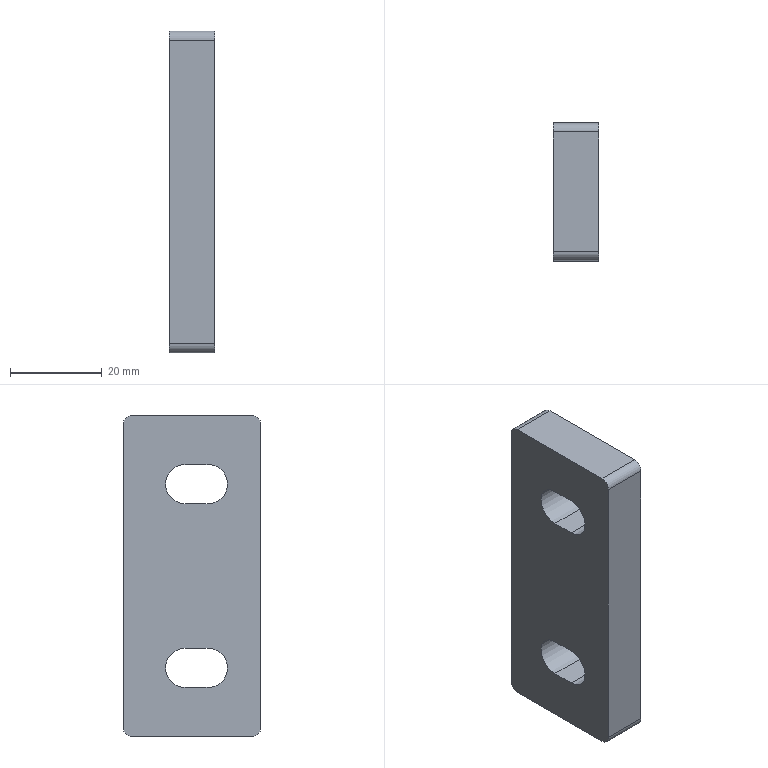Component | SolidWorks | BladeHolderPlate.1-2 | 1 solid | 26 faces | box 10 x 30 x 70 mm | volume 18626 mm3 | cylinder 12 | plane 10 | cone 4 | commonest cylinder face diameters 4.2 x4 4 x4 8.5 x4
build123d program:
from build123d import *

# Parameters (mm, degrees)
BOSS_EXTRUDE1_DEPTH   = 10
M5_TAPPED_HOLE1_D     = 4.2
M5_TAPPED_HOLE1_DEPTH = 12.4
M5_TAPPED_HOLE1_TIP   = 1.262
CUT_EXTRUDE1_DEPTH    = 15


with BuildPart() as part:
    # Sketch1 → Boss-Extrude1 (new body)
    with BuildSketch(Plane.XY):
        with BuildLine():
            Line((-33, 15), (33, 15))
            ThreePointArc((33, 15), (34.414, 14.414), (35, 13))
            Line((35, 13), (35, -13))
            ThreePointArc((35, -13), (34.414, -14.414), (33, -15))
            Line((33, -15), (-33, -15))
            ThreePointArc((-33, -15), (-34.414, -14.414), (-35, -13))
            Line((-35, -13), (-35, 13))
            ThreePointArc((-35, 13), (-34.414, 14.414), (-33, 15))
        make_face()
    extrude(amount=BOSS_EXTRUDE1_DEPTH)

    # M5 Tapped Hole1
    with Locations(Plane(origin=(0, 15, 0), x_dir=(-1, 0, 0), z_dir=(0, 1, 0))):
        with Locations((27.5, 5), (-27.5, 5)):
            Hole(M5_TAPPED_HOLE1_D / 2, depth=M5_TAPPED_HOLE1_DEPTH)
            with Locations((0, 0, -(M5_TAPPED_HOLE1_DEPTH + M5_TAPPED_HOLE1_TIP / 2))):  # 118° drill point
                Cone(0, M5_TAPPED_HOLE1_D / 2, M5_TAPPED_HOLE1_TIP, mode=Mode.SUBTRACT)

    # Sketch5 → Cut-Extrude1 (cut)
    with BuildSketch(Plane.XY.offset(10)):
        with BuildLine():
            Line((-15.75, 1.5), (-15.75, -3.5))
            ThreePointArc((-15.75, -3.5), (-20, -7.75), (-24.25, -3.5))
            Line((-24.25, -3.5), (-24.25, 1.5))
            ThreePointArc((-24.25, 1.5), (-20, 5.75), (-15.75, 1.5))
        make_face()
        with BuildLine():
            Line((24.25, 1.5), (24.25, -3.5))
            ThreePointArc((24.25, -3.5), (20, -7.75), (15.75, -3.5))
            Line((15.75, -3.5), (15.75, 1.5))
            ThreePointArc((15.75, 1.5), (20, 5.75), (24.25, 1.5))
        make_face()
    extrude(amount=-CUT_EXTRUDE1_DEPTH, mode=Mode.SUBTRACT)


solid = part.part

# Placed as in the assembly
solid = solid.moved(Location((-27.75, 191, 0), (0, 90, 0)))
STEP:
#1=CARTESIAN_POINT('',(-0.813,7.622,-1.083));
#2=VERTEX_POINT('',#1);
#3=CARTESIAN_POINT('',(-0.9783,7.622,-1.083));
#4=VERTEX_POINT('',#3);
#5=CARTESIAN_POINT('',(-0.8957,7.622,-1.083));
#6=DIRECTION('',(-0.,1.,-0.));
#7=DIRECTION('',(-1.,0.,0.));
#8=AXIS2_PLACEMENT_3D('',#5,#6,#7);
#9=CIRCLE('',#8,0.08268);
#10=EDGE_CURVE('',#2,#4,#9,.T.);
#11=ORIENTED_EDGE('',*,*,#10,.F.);
#12=CARTESIAN_POINT('',(-0.813,8.11,-1.083));
#13=VERTEX_POINT('',#12);
#14=CARTESIAN_POINT('',(-0.813,8.11,-1.083));
#15=DIRECTION('',(-0.,1.,-0.));
#16=VECTOR('',#15,39.37);
#17=LINE('',#14,#16);
#18=EDGE_CURVE('',#2,#13,#17,.T.);
#19=ORIENTED_EDGE('',*,*,#18,.T.);
#20=CARTESIAN_POINT('',(-0.9783,8.11,-1.083));
#21=VERTEX_POINT('',#20);
#22=CARTESIAN_POINT('',(-0.8957,8.11,-1.083));
#23=DIRECTION('',(-0.,1.,-0.));
#24=DIRECTION('',(-1.,0.,0.));
#25=AXIS2_PLACEMENT_3D('',#22,#23,#24);
#26=CIRCLE('',#25,0.08268);
#27=EDGE_CURVE('',#13,#21,#26,.T.);
#28=ORIENTED_EDGE('',*,*,#27,.T.);
#29=CARTESIAN_POINT('',(-0.9783,8.11,-1.083));
#30=DIRECTION('',(-0.,1.,-0.));
#31=VECTOR('',#30,39.37);
#32=LINE('',#29,#31);
#33=EDGE_CURVE('',#4,#21,#32,.T.);
#34=ORIENTED_EDGE('',*,*,#33,.F.);
#35=EDGE_LOOP('',(#11,#19,#28,#34));
#36=FACE_OUTER_BOUND('',#35,.T.);
#37=CARTESIAN_POINT('',(-0.8957,8.11,-1.083));
#38=DIRECTION('',(-0.,1.,-0.));
#39=DIRECTION('',(-1.,0.,0.));
#40=AXIS2_PLACEMENT_3D('',#37,#38,#39);
#41=CYLINDRICAL_SURFACE('',#40,0.08268);
#42=ADVANCED_FACE('',(#36),#41,.F.);
#43=CARTESIAN_POINT('',(-0.8957,7.572,-1.083));
#44=VERTEX_POINT('',#43);
#45=CARTESIAN_POINT('',(-0.9783,7.622,-1.083));
#46=DIRECTION('',(-0.8572,0.515,0.));
#47=VECTOR('',#46,39.37);
#48=LINE('',#45,#47);
#49=EDGE_CURVE('',#44,#4,#48,.T.);
#50=ORIENTED_EDGE('',*,*,#49,.F.);
#51=CARTESIAN_POINT('',(-0.813,7.622,-1.083));
#52=DIRECTION('',(0.8572,0.515,0.));
#53=VECTOR('',#52,39.37);
#54=LINE('',#51,#53);
#55=EDGE_CURVE('',#44,#2,#54,.T.);
#56=ORIENTED_EDGE('',*,*,#55,.T.);
#57=ORIENTED_EDGE('',*,*,#10,.T.);
#58=EDGE_LOOP('',(#50,#56,#57));
#59=FACE_OUTER_BOUND('',#58,.T.);
#60=CARTESIAN_POINT('',(-0.8957,7.622,-1.083));
#61=DIRECTION('',(-0.,1.,-0.));
#62=DIRECTION('',(-1.,0.,0.));
#63=AXIS2_PLACEMENT_3D('',#60,#61,#62);
#64=CONICAL_SURFACE('',#63,0.08268,1.03);
#65=ADVANCED_FACE('',(#59),#64,.F.);
#66=CARTESIAN_POINT('',(-0.813,7.622,1.083));
#67=VERTEX_POINT('',#66);
#68=CARTESIAN_POINT('',(-0.9783,7.622,1.083));
#69=VERTEX_POINT('',#68);
#70=CARTESIAN_POINT('',(-0.8957,7.622,1.083));
#71=DIRECTION('',(-0.,1.,-0.));
#72=DIRECTION('',(-1.,0.,0.));
#73=AXIS2_PLACEMENT_3D('',#70,#71,#72);
#74=CIRCLE('',#73,0.08268);
#75=EDGE_CURVE('',#67,#69,#74,.T.);
#76=ORIENTED_EDGE('',*,*,#75,.F.);
#77=CARTESIAN_POINT('',(-0.813,8.11,1.083));
#78=VERTEX_POINT('',#77);
#79=CARTESIAN_POINT('',(-0.813,8.11,1.083));
#80=DIRECTION('',(-0.,1.,-0.));
#81=VECTOR('',#80,39.37);
#82=LINE('',#79,#81);
#83=EDGE_CURVE('',#67,#78,#82,.T.);
#84=ORIENTED_EDGE('',*,*,#83,.T.);
#85=CARTESIAN_POINT('',(-0.9783,8.11,1.083));
#86=VERTEX_POINT('',#85);
#87=CARTESIAN_POINT('',(-0.8957,8.11,1.083));
#88=DIRECTION('',(-0.,1.,-0.));
#89=DIRECTION('',(-1.,0.,0.));
#90=AXIS2_PLACEMENT_3D('',#87,#88,#89);
#91=CIRCLE('',#90,0.08268);
#92=EDGE_CURVE('',#78,#86,#91,.T.);
#93=ORIENTED_EDGE('',*,*,#92,.T.);
#94=CARTESIAN_POINT('',(-0.9783,8.11,1.083));
#95=DIRECTION('',(-0.,1.,-0.));
#96=VECTOR('',#95,39.37);
#97=LINE('',#94,#96);
#98=EDGE_CURVE('',#69,#86,#97,.T.);
#99=ORIENTED_EDGE('',*,*,#98,.F.);
#100=EDGE_LOOP('',(#76,#84,#93,#99));
#101=FACE_OUTER_BOUND('',#100,.T.);
#102=CARTESIAN_POINT('',(-0.8957,8.11,1.083));
#103=DIRECTION('',(-0.,1.,-0.));
#104=DIRECTION('',(-1.,0.,0.));
#105=AXIS2_PLACEMENT_3D('',#102,#103,#104);
#106=CYLINDRICAL_SURFACE('',#105,0.08268);
#107=ADVANCED_FACE('',(#101),#106,.F.);
#108=CARTESIAN_POINT('',(-0.8957,7.572,1.083));
#109=VERTEX_POINT('',#108);
#110=CARTESIAN_POINT('',(-0.9783,7.622,1.083));
#111=DIRECTION('',(-0.8572,0.515,0.));
#112=VECTOR('',#111,39.37);
#113=LINE('',#110,#112);
#114=EDGE_CURVE('',#109,#69,#113,.T.);
#115=ORIENTED_EDGE('',*,*,#114,.F.);
#116=CARTESIAN_POINT('',(-0.813,7.622,1.083));
#117=DIRECTION('',(0.8572,0.515,0.));
#118=VECTOR('',#117,39.37);
#119=LINE('',#116,#118);
#120=EDGE_CURVE('',#109,#67,#119,.T.);
#121=ORIENTED_EDGE('',*,*,#120,.T.);
#122=ORIENTED_EDGE('',*,*,#75,.T.);
#123=EDGE_LOOP('',(#115,#121,#122));
#124=FACE_OUTER_BOUND('',#123,.T.);
#125=CARTESIAN_POINT('',(-0.8957,7.622,1.083));
#126=DIRECTION('',(-0.,1.,-0.));
#127=DIRECTION('',(-1.,0.,0.));
#128=AXIS2_PLACEMENT_3D('',#125,#126,#127);
#129=CONICAL_SURFACE('',#128,0.08268,1.03);
#130=ADVANCED_FACE('',(#124),#129,.F.);
#131=CARTESIAN_POINT('',(-0.6988,7.008,-1.378));
#132=VERTEX_POINT('',#131);
#133=CARTESIAN_POINT('',(-0.6988,6.929,-1.299));
#134=VERTEX_POINT('',#133);
#135=CARTESIAN_POINT('',(-0.6988,7.008,-1.299));
#136=DIRECTION('',(-1.,-0.,0.));
#137=DIRECTION('',(0.,0.,1.));
#138=AXIS2_PLACEMENT_3D('',#135,#136,#137);
#139=CIRCLE('',#138,0.07874);
#140=EDGE_CURVE('',#132,#134,#139,.T.);
#141=ORIENTED_EDGE('',*,*,#140,.T.);
#142=CARTESIAN_POINT('',(-1.093,6.929,-1.299));
#143=VERTEX_POINT('',#142);
#144=CARTESIAN_POINT('',(-1.093,6.929,-1.299));
#145=DIRECTION('',(1.,0.,-0.));
#146=VECTOR('',#145,39.37);
#147=LINE('',#144,#146);
#148=EDGE_CURVE('',#143,#134,#147,.T.);
#149=ORIENTED_EDGE('',*,*,#148,.F.);
#150=CARTESIAN_POINT('',(-1.093,7.008,-1.378));
#151=VERTEX_POINT('',#150);
#152=CARTESIAN_POINT('',(-1.093,7.008,-1.299));
#153=DIRECTION('',(-1.,-0.,0.));
#154=DIRECTION('',(0.,0.,1.));
#155=AXIS2_PLACEMENT_3D('',#152,#153,#154);
#156=CIRCLE('',#155,0.07874);
#157=EDGE_CURVE('',#151,#143,#156,.T.);
#158=ORIENTED_EDGE('',*,*,#157,.F.);
#159=CARTESIAN_POINT('',(-1.093,7.008,-1.378));
#160=DIRECTION('',(1.,0.,-0.));
#161=VECTOR('',#160,39.37);
#162=LINE('',#159,#161);
#163=EDGE_CURVE('',#151,#132,#162,.T.);
#164=ORIENTED_EDGE('',*,*,#163,.T.);
#165=EDGE_LOOP('',(#141,#149,#158,#164));
#166=FACE_OUTER_BOUND('',#165,.T.);
#167=CARTESIAN_POINT('',(-1.093,7.008,-1.299));
#168=DIRECTION('',(1.,0.,-0.));
#169=DIRECTION('',(0.,0.,-1.));
#170=AXIS2_PLACEMENT_3D('',#167,#168,#169);
#171=CYLINDRICAL_SURFACE('',#170,0.07874);
#172=ADVANCED_FACE('',(#166),#171,.T.);
#173=CARTESIAN_POINT('',(-0.6988,6.929,1.299));
#174=VERTEX_POINT('',#173);
#175=CARTESIAN_POINT('',(-0.6988,6.929,-1.299));
#176=DIRECTION('',(0.,0.,1.));
#177=VECTOR('',#176,39.37);
#178=LINE('',#175,#177);
#179=EDGE_CURVE('',#134,#174,#178,.T.);
#180=ORIENTED_EDGE('',*,*,#179,.T.);
#181=CARTESIAN_POINT('',(-1.093,6.929,1.299));
#182=VERTEX_POINT('',#181);
#183=CARTESIAN_POINT('',(-1.093,6.929,1.299));
#184=DIRECTION('',(1.,0.,-0.));
#185=VECTOR('',#184,39.37);
#186=LINE('',#183,#185);
#187=EDGE_CURVE('',#182,#174,#186,.T.);
#188=ORIENTED_EDGE('',*,*,#187,.F.);
#189=CARTESIAN_POINT('',(-1.093,6.929,-1.299));
#190=DIRECTION('',(0.,0.,1.));
#191=VECTOR('',#190,39.37);
#192=LINE('',#189,#191);
#193=EDGE_CURVE('',#143,#182,#192,.T.);
#194=ORIENTED_EDGE('',*,*,#193,.F.);
#195=ORIENTED_EDGE('',*,*,#148,.T.);
#196=EDGE_LOOP('',(#180,#188,#194,#195));
#197=FACE_OUTER_BOUND('',#196,.T.);
#198=CARTESIAN_POINT('',(-1.093,6.929,-1.299));
#199=DIRECTION('',(-0.,1.,-0.));
#200=DIRECTION('',(-0.,-0.,-1.));
#201=AXIS2_PLACEMENT_3D('',#198,#199,#200);
#202=PLANE('',#201);
#203=ADVANCED_FACE('',(#197),#202,.F.);
#204=CARTESIAN_POINT('',(-0.6988,7.008,1.378));
#205=VERTEX_POINT('',#204);
#206=CARTESIAN_POINT('',(-0.6988,7.008,1.299));
#207=DIRECTION('',(-1.,-0.,0.));
#208=DIRECTION('',(0.,0.,1.));
#209=AXIS2_PLACEMENT_3D('',#206,#207,#208);
#210=CIRCLE('',#209,0.07874);
#211=EDGE_CURVE('',#174,#205,#210,.T.);
#212=ORIENTED_EDGE('',*,*,#211,.T.);
#213=CARTESIAN_POINT('',(-1.093,7.008,1.378));
#214=VERTEX_POINT('',#213);
#215=CARTESIAN_POINT('',(-1.093,7.008,1.378));
#216=DIRECTION('',(1.,0.,-0.));
#217=VECTOR('',#216,39.37);
#218=LINE('',#215,#217);
#219=EDGE_CURVE('',#214,#205,#218,.T.);
#220=ORIENTED_EDGE('',*,*,#219,.F.);
#221=CARTESIAN_POINT('',(-1.093,7.008,1.299));
#222=DIRECTION('',(-1.,-0.,0.));
#223=DIRECTION('',(0.,0.,1.));
#224=AXIS2_PLACEMENT_3D('',#221,#222,#223);
#225=CIRCLE('',#224,0.07874);
#226=EDGE_CURVE('',#182,#214,#225,.T.);
#227=ORIENTED_EDGE('',*,*,#226,.F.);
#228=ORIENTED_EDGE('',*,*,#187,.T.);
#229=EDGE_LOOP('',(#212,#220,#227,#228));
#230=FACE_OUTER_BOUND('',#229,.T.);
#231=CARTESIAN_POINT('',(-1.093,7.008,1.299));
#232=DIRECTION('',(1.,0.,-0.));
#233=DIRECTION('',(0.,0.,-1.));
#234=AXIS2_PLACEMENT_3D('',#231,#232,#233);
#235=CYLINDRICAL_SURFACE('',#234,0.07874);
#236=ADVANCED_FACE('',(#230),#235,.T.);
#237=CARTESIAN_POINT('',(-0.6988,8.031,1.378));
#238=VERTEX_POINT('',#237);
#239=CARTESIAN_POINT('',(-0.6988,8.031,1.378));
#240=DIRECTION('',(-0.,1.,-0.));
#241=VECTOR('',#240,39.37);
#242=LINE('',#239,#241);
#243=EDGE_CURVE('',#205,#238,#242,.T.);
#244=ORIENTED_EDGE('',*,*,#243,.T.);
#245=CARTESIAN_POINT('',(-1.093,8.031,1.378));
#246=VERTEX_POINT('',#245);
#247=CARTESIAN_POINT('',(-1.093,8.031,1.378));
#248=DIRECTION('',(1.,0.,-0.));
#249=VECTOR('',#248,39.37);
#250=LINE('',#247,#249);
#251=EDGE_CURVE('',#246,#238,#250,.T.);
#252=ORIENTED_EDGE('',*,*,#251,.F.);
#253=CARTESIAN_POINT('',(-1.093,8.031,1.378));
#254=DIRECTION('',(-0.,1.,-0.));
#255=VECTOR('',#254,39.37);
#256=LINE('',#253,#255);
#257=EDGE_CURVE('',#214,#246,#256,.T.);
#258=ORIENTED_EDGE('',*,*,#257,.F.);
#259=ORIENTED_EDGE('',*,*,#219,.T.);
#260=EDGE_LOOP('',(#244,#252,#258,#259));
#261=FACE_OUTER_BOUND('',#260,.T.);
#262=CARTESIAN_POINT('',(-1.093,8.031,1.378));
#263=DIRECTION('',(-0.,-0.,-1.));
#264=DIRECTION('',(-1.,-0.,0.));
#265=AXIS2_PLACEMENT_3D('',#262,#263,#264);
#266=PLANE('',#265);
#267=ADVANCED_FACE('',(#261),#266,.F.);
#268=CARTESIAN_POINT('',(-0.6988,8.11,1.299));
#269=VERTEX_POINT('',#268);
#270=CARTESIAN_POINT('',(-0.6988,8.031,1.299));
#271=DIRECTION('',(-1.,-0.,0.));
#272=DIRECTION('',(0.,0.,1.));
#273=AXIS2_PLACEMENT_3D('',#270,#271,#272);
#274=CIRCLE('',#273,0.07874);
#275=EDGE_CURVE('',#238,#269,#274,.T.);
#276=ORIENTED_EDGE('',*,*,#275,.T.);
#277=CARTESIAN_POINT('',(-1.093,8.11,1.299));
#278=VERTEX_POINT('',#277);
#279=CARTESIAN_POINT('',(-1.093,8.11,1.299));
#280=DIRECTION('',(1.,0.,-0.));
#281=VECTOR('',#280,39.37);
#282=LINE('',#279,#281);
#283=EDGE_CURVE('',#278,#269,#282,.T.);
#284=ORIENTED_EDGE('',*,*,#283,.F.);
#285=CARTESIAN_POINT('',(-1.093,8.031,1.299));
#286=DIRECTION('',(-1.,-0.,0.));
#287=DIRECTION('',(0.,0.,1.));
#288=AXIS2_PLACEMENT_3D('',#285,#286,#287);
#289=CIRCLE('',#288,0.07874);
#290=EDGE_CURVE('',#246,#278,#289,.T.);
#291=ORIENTED_EDGE('',*,*,#290,.F.);
#292=ORIENTED_EDGE('',*,*,#251,.T.);
#293=EDGE_LOOP('',(#276,#284,#291,#292));
#294=FACE_OUTER_BOUND('',#293,.T.);
#295=CARTESIAN_POINT('',(-1.093,8.031,1.299));
#296=DIRECTION('',(1.,0.,-0.));
#297=DIRECTION('',(0.,0.,-1.));
#298=AXIS2_PLACEMENT_3D('',#295,#296,#297);
#299=CYLINDRICAL_SURFACE('',#298,0.07874);
#300=ADVANCED_FACE('',(#294),#299,.T.);
#301=CARTESIAN_POINT('',(-0.8957,8.11,-1.083));
#302=DIRECTION('',(-0.,1.,-0.));
#303=DIRECTION('',(-1.,0.,0.));
#304=AXIS2_PLACEMENT_3D('',#301,#302,#303);
#305=CIRCLE('',#304,0.08268);
#306=EDGE_CURVE('',#21,#13,#305,.T.);
#307=ORIENTED_EDGE('',*,*,#306,.F.);
#308=ORIENTED_EDGE('',*,*,#27,.F.);
#309=EDGE_LOOP('',(#307,#308));
#310=FACE_BOUND('',#309,.T.);
#311=CARTESIAN_POINT('',(-0.8957,8.11,1.083));
#312=DIRECTION('',(-0.,1.,-0.));
#313=DIRECTION('',(-1.,0.,0.));
#314=AXIS2_PLACEMENT_3D('',#311,#312,#313);
#315=CIRCLE('',#314,0.08268);
#316=EDGE_CURVE('',#86,#78,#315,.T.);
#317=ORIENTED_EDGE('',*,*,#316,.F.);
#318=ORIENTED_EDGE('',*,*,#92,.F.);
#319=EDGE_LOOP('',(#317,#318));
#320=FACE_BOUND('',#319,.T.);
#321=CARTESIAN_POINT('',(-0.6988,8.11,-1.299));
#322=VERTEX_POINT('',#321);
#323=CARTESIAN_POINT('',(-0.6988,8.11,-1.299));
#324=DIRECTION('',(-0.,-0.,-1.));
#325=VECTOR('',#324,39.37);
#326=LINE('',#323,#325);
#327=EDGE_CURVE('',#269,#322,#326,.T.);
#328=ORIENTED_EDGE('',*,*,#327,.T.);
#329=CARTESIAN_POINT('',(-1.093,8.11,-1.299));
#330=VERTEX_POINT('',#329);
#331=CARTESIAN_POINT('',(-1.093,8.11,-1.299));
#332=DIRECTION('',(1.,0.,-0.));
#333=VECTOR('',#332,39.37);
#334=LINE('',#331,#333);
#335=EDGE_CURVE('',#330,#322,#334,.T.);
#336=ORIENTED_EDGE('',*,*,#335,.F.);
#337=CARTESIAN_POINT('',(-1.093,8.11,-1.299));
#338=DIRECTION('',(-0.,-0.,-1.));
#339=VECTOR('',#338,39.37);
#340=LINE('',#337,#339);
#341=EDGE_CURVE('',#278,#330,#340,.T.);
#342=ORIENTED_EDGE('',*,*,#341,.F.);
#343=ORIENTED_EDGE('',*,*,#283,.T.);
#344=EDGE_LOOP('',(#328,#336,#342,#343));
#345=FACE_OUTER_BOUND('',#344,.T.);
#346=CARTESIAN_POINT('',(-1.093,8.11,-1.299));
#347=DIRECTION('',(0.,-1.,0.));
#348=DIRECTION('',(0.,0.,1.));
#349=AXIS2_PLACEMENT_3D('',#346,#347,#348);
#350=PLANE('',#349);
#351=ADVANCED_FACE('',(#310,#320,#345),#350,.F.);
#352=CARTESIAN_POINT('',(-0.6988,8.031,-1.378));
#353=VERTEX_POINT('',#352);
#354=CARTESIAN_POINT('',(-0.6988,8.031,-1.299));
#355=DIRECTION('',(-1.,-0.,0.));
#356=DIRECTION('',(0.,0.,1.));
#357=AXIS2_PLACEMENT_3D('',#354,#355,#356);
#358=CIRCLE('',#357,0.07874);
#359=EDGE_CURVE('',#322,#353,#358,.T.);
#360=ORIENTED_EDGE('',*,*,#359,.T.);
#361=CARTESIAN_POINT('',(-1.093,8.031,-1.378));
#362=VERTEX_POINT('',#361);
#363=CARTESIAN_POINT('',(-1.093,8.031,-1.378));
#364=DIRECTION('',(1.,0.,-0.));
#365=VECTOR('',#364,39.37);
#366=LINE('',#363,#365);
#367=EDGE_CURVE('',#362,#353,#366,.T.);
#368=ORIENTED_EDGE('',*,*,#367,.F.);
#369=CARTESIAN_POINT('',(-1.093,8.031,-1.299));
#370=DIRECTION('',(-1.,-0.,0.));
#371=DIRECTION('',(0.,0.,1.));
#372=AXIS2_PLACEMENT_3D('',#369,#370,#371);
#373=CIRCLE('',#372,0.07874);
#374=EDGE_CURVE('',#330,#362,#373,.T.);
#375=ORIENTED_EDGE('',*,*,#374,.F.);
#376=ORIENTED_EDGE('',*,*,#335,.T.);
#377=EDGE_LOOP('',(#360,#368,#375,#376));
#378=FACE_OUTER_BOUND('',#377,.T.);
#379=CARTESIAN_POINT('',(-1.093,8.031,-1.299));
#380=DIRECTION('',(1.,0.,-0.));
#381=DIRECTION('',(0.,0.,-1.));
#382=AXIS2_PLACEMENT_3D('',#379,#380,#381);
#383=CYLINDRICAL_SURFACE('',#382,0.07874);
#384=ADVANCED_FACE('',(#378),#383,.T.);
#385=CARTESIAN_POINT('',(-0.6988,8.031,-1.378));
#386=DIRECTION('',(0.,-1.,0.));
#387=VECTOR('',#386,39.37);
#388=LINE('',#385,#387);
#389=EDGE_CURVE('',#353,#132,#388,.T.);
#390=ORIENTED_EDGE('',*,*,#389,.T.);
#391=ORIENTED_EDGE('',*,*,#163,.F.);
#392=CARTESIAN_POINT('',(-1.093,8.031,-1.378));
#393=DIRECTION('',(0.,-1.,0.));
#394=VECTOR('',#393,39.37);
#395=LINE('',#392,#394);
#396=EDGE_CURVE('',#362,#151,#395,.T.);
#397=ORIENTED_EDGE('',*,*,#396,.F.);
#398=ORIENTED_EDGE('',*,*,#367,.T.);
#399=EDGE_LOOP('',(#390,#391,#397,#398));
#400=FACE_OUTER_BOUND('',#399,.T.);
#401=CARTESIAN_POINT('',(-1.093,8.031,-1.378));
#402=DIRECTION('',(0.,0.,1.));
#403=DIRECTION('',(1.,0.,-0.));
#404=AXIS2_PLACEMENT_3D('',#401,#402,#403);
#405=PLANE('',#404);
#406=ADVANCED_FACE('',(#400),#405,.F.);
#407=CARTESIAN_POINT('',(-1.093,7.579,0.9547));
#408=VERTEX_POINT('',#407);
#409=CARTESIAN_POINT('',(-1.093,7.579,0.6201));
#410=VERTEX_POINT('',#409);
#411=CARTESIAN_POINT('',(-1.093,7.579,0.7874));
#412=DIRECTION('',(-1.,-0.,0.));
#413=DIRECTION('',(0.,0.,1.));
#414=AXIS2_PLACEMENT_3D('',#411,#412,#413);
#415=CIRCLE('',#414,0.1673);
#416=EDGE_CURVE('',#408,#410,#415,.T.);
#417=ORIENTED_EDGE('',*,*,#416,.F.);
#418=CARTESIAN_POINT('',(-1.093,7.382,0.9547));
#419=VERTEX_POINT('',#418);
#420=CARTESIAN_POINT('',(-1.093,7.579,0.9547));
#421=DIRECTION('',(-0.,1.,-0.));
#422=VECTOR('',#421,39.37);
#423=LINE('',#420,#422);
#424=EDGE_CURVE('',#419,#408,#423,.T.);
#425=ORIENTED_EDGE('',*,*,#424,.F.);
#426=CARTESIAN_POINT('',(-1.093,7.382,0.6201));
#427=VERTEX_POINT('',#426);
#428=CARTESIAN_POINT('',(-1.093,7.382,0.7874));
#429=DIRECTION('',(-1.,-0.,0.));
#430=DIRECTION('',(0.,0.,1.));
#431=AXIS2_PLACEMENT_3D('',#428,#429,#430);
#432=CIRCLE('',#431,0.1673);
#433=EDGE_CURVE('',#427,#419,#432,.T.);
#434=ORIENTED_EDGE('',*,*,#433,.F.);
#435=CARTESIAN_POINT('',(-1.093,7.579,0.6201));
#436=DIRECTION('',(0.,-1.,0.));
#437=VECTOR('',#436,39.37);
#438=LINE('',#435,#437);
#439=EDGE_CURVE('',#410,#427,#438,.T.);
#440=ORIENTED_EDGE('',*,*,#439,.F.);
#441=EDGE_LOOP('',(#417,#425,#434,#440));
#442=FACE_BOUND('',#441,.T.);
#443=CARTESIAN_POINT('',(-1.093,7.579,-0.6201));
#444=VERTEX_POINT('',#443);
#445=CARTESIAN_POINT('',(-1.093,7.579,-0.9547));
#446=VERTEX_POINT('',#445);
#447=CARTESIAN_POINT('',(-1.093,7.579,-0.7874));
#448=DIRECTION('',(-1.,-0.,0.));
#449=DIRECTION('',(0.,0.,1.));
#450=AXIS2_PLACEMENT_3D('',#447,#448,#449);
#451=CIRCLE('',#450,0.1673);
#452=EDGE_CURVE('',#444,#446,#451,.T.);
#453=ORIENTED_EDGE('',*,*,#452,.F.);
#454=CARTESIAN_POINT('',(-1.093,7.382,-0.6201));
#455=VERTEX_POINT('',#454);
#456=CARTESIAN_POINT('',(-1.093,7.579,-0.6201));
#457=DIRECTION('',(-0.,1.,-0.));
#458=VECTOR('',#457,39.37);
#459=LINE('',#456,#458);
#460=EDGE_CURVE('',#455,#444,#459,.T.);
#461=ORIENTED_EDGE('',*,*,#460,.F.);
#462=CARTESIAN_POINT('',(-1.093,7.382,-0.9547));
#463=VERTEX_POINT('',#462);
#464=CARTESIAN_POINT('',(-1.093,7.382,-0.7874));
#465=DIRECTION('',(-1.,-0.,0.));
#466=DIRECTION('',(0.,0.,1.));
#467=AXIS2_PLACEMENT_3D('',#464,#465,#466);
#468=CIRCLE('',#467,0.1673);
#469=EDGE_CURVE('',#463,#455,#468,.T.);
#470=ORIENTED_EDGE('',*,*,#469,.F.);
#471=CARTESIAN_POINT('',(-1.093,7.579,-0.9547));
#472=DIRECTION('',(0.,-1.,0.));
#473=VECTOR('',#472,39.37);
#474=LINE('',#471,#473);
#475=EDGE_CURVE('',#446,#463,#474,.T.);
#476=ORIENTED_EDGE('',*,*,#475,.F.);
#477=EDGE_LOOP('',(#453,#461,#470,#476));
#478=FACE_BOUND('',#477,.T.);
#479=ORIENTED_EDGE('',*,*,#157,.T.);
#480=ORIENTED_EDGE('',*,*,#193,.T.);
#481=ORIENTED_EDGE('',*,*,#226,.T.);
#482=ORIENTED_EDGE('',*,*,#257,.T.);
#483=ORIENTED_EDGE('',*,*,#290,.T.);
#484=ORIENTED_EDGE('',*,*,#341,.T.);
#485=ORIENTED_EDGE('',*,*,#374,.T.);
#486=ORIENTED_EDGE('',*,*,#396,.T.);
#487=EDGE_LOOP('',(#479,#480,#481,#482,#483,#484,#485,#486));
#488=FACE_OUTER_BOUND('',#487,.T.);
#489=CARTESIAN_POINT('',(-1.093,7.008,-1.299));
#490=DIRECTION('',(-1.,-0.,0.));
#491=DIRECTION('',(0.,0.,1.));
#492=AXIS2_PLACEMENT_3D('',#489,#490,#491);
#493=PLANE('',#492);
#494=ADVANCED_FACE('',(#442,#478,#488),#493,.T.);
#495=CARTESIAN_POINT('',(-0.6988,7.382,0.9547));
#496=VERTEX_POINT('',#495);
#497=CARTESIAN_POINT('',(-0.6988,7.579,0.9547));
#498=VERTEX_POINT('',#497);
#499=CARTESIAN_POINT('',(-0.6988,7.008,0.9547));
#500=DIRECTION('',(-0.,1.,-0.));
#501=VECTOR('',#500,39.37);
#502=LINE('',#499,#501);
#503=EDGE_CURVE('',#496,#498,#502,.T.);
#504=ORIENTED_EDGE('',*,*,#503,.T.);
#505=CARTESIAN_POINT('',(-0.6988,7.579,0.6201));
#506=VERTEX_POINT('',#505);
#507=CARTESIAN_POINT('',(-0.6988,7.579,0.7874));
#508=DIRECTION('',(-1.,-0.,0.));
#509=DIRECTION('',(0.,0.,1.));
#510=AXIS2_PLACEMENT_3D('',#507,#508,#509);
#511=CIRCLE('',#510,0.1673);
#512=EDGE_CURVE('',#498,#506,#511,.T.);
#513=ORIENTED_EDGE('',*,*,#512,.T.);
#514=CARTESIAN_POINT('',(-0.6988,7.382,0.6201));
#515=VERTEX_POINT('',#514);
#516=CARTESIAN_POINT('',(-0.6988,7.008,0.6201));
#517=DIRECTION('',(0.,-1.,0.));
#518=VECTOR('',#517,39.37);
#519=LINE('',#516,#518);
#520=EDGE_CURVE('',#506,#515,#519,.T.);
#521=ORIENTED_EDGE('',*,*,#520,.T.);
#522=CARTESIAN_POINT('',(-0.6988,7.382,0.7874));
#523=DIRECTION('',(-1.,-0.,0.));
#524=DIRECTION('',(0.,0.,1.));
#525=AXIS2_PLACEMENT_3D('',#522,#523,#524);
#526=CIRCLE('',#525,0.1673);
#527=EDGE_CURVE('',#515,#496,#526,.T.);
#528=ORIENTED_EDGE('',*,*,#527,.T.);
#529=EDGE_LOOP('',(#504,#513,#521,#528));
#530=FACE_BOUND('',#529,.T.);
#531=CARTESIAN_POINT('',(-0.6988,7.382,-0.6201));
#532=VERTEX_POINT('',#531);
#533=CARTESIAN_POINT('',(-0.6988,7.579,-0.6201));
#534=VERTEX_POINT('',#533);
#535=CARTESIAN_POINT('',(-0.6988,7.008,-0.6201));
#536=DIRECTION('',(-0.,1.,-0.));
#537=VECTOR('',#536,39.37);
#538=LINE('',#535,#537);
#539=EDGE_CURVE('',#532,#534,#538,.T.);
#540=ORIENTED_EDGE('',*,*,#539,.T.);
#541=CARTESIAN_POINT('',(-0.6988,7.579,-0.9547));
#542=VERTEX_POINT('',#541);
#543=CARTESIAN_POINT('',(-0.6988,7.579,-0.7874));
#544=DIRECTION('',(-1.,-0.,0.));
#545=DIRECTION('',(0.,0.,1.));
#546=AXIS2_PLACEMENT_3D('',#543,#544,#545);
#547=CIRCLE('',#546,0.1673);
#548=EDGE_CURVE('',#534,#542,#547,.T.);
#549=ORIENTED_EDGE('',*,*,#548,.T.);
#550=CARTESIAN_POINT('',(-0.6988,7.382,-0.9547));
#551=VERTEX_POINT('',#550);
#552=CARTESIAN_POINT('',(-0.6988,7.008,-0.9547));
#553=DIRECTION('',(0.,-1.,0.));
#554=VECTOR('',#553,39.37);
#555=LINE('',#552,#554);
#556=EDGE_CURVE('',#542,#551,#555,.T.);
#557=ORIENTED_EDGE('',*,*,#556,.T.);
#558=CARTESIAN_POINT('',(-0.6988,7.382,-0.7874));
#559=DIRECTION('',(-1.,-0.,0.));
#560=DIRECTION('',(0.,0.,1.));
#561=AXIS2_PLACEMENT_3D('',#558,#559,#560);
#562=CIRCLE('',#561,0.1673);
#563=EDGE_CURVE('',#551,#532,#562,.T.);
#564=ORIENTED_EDGE('',*,*,#563,.T.);
#565=EDGE_LOOP('',(#540,#549,#557,#564));
#566=FACE_BOUND('',#565,.T.);
#567=ORIENTED_EDGE('',*,*,#140,.F.);
#568=ORIENTED_EDGE('',*,*,#389,.F.);
#569=ORIENTED_EDGE('',*,*,#359,.F.);
#570=ORIENTED_EDGE('',*,*,#327,.F.);
#571=ORIENTED_EDGE('',*,*,#275,.F.);
#572=ORIENTED_EDGE('',*,*,#243,.F.);
#573=ORIENTED_EDGE('',*,*,#211,.F.);
#574=ORIENTED_EDGE('',*,*,#179,.F.);
#575=EDGE_LOOP('',(#567,#568,#569,#570,#571,#572,#573,#574));
#576=FACE_OUTER_BOUND('',#575,.T.);
#577=CARTESIAN_POINT('',(-0.6988,7.008,-1.299));
#578=DIRECTION('',(-1.,-0.,0.));
#579=DIRECTION('',(0.,0.,1.));
#580=AXIS2_PLACEMENT_3D('',#577,#578,#579);
#581=PLANE('',#580);
#582=ADVANCED_FACE('',(#530,#566,#576),#581,.F.);
#583=ORIENTED_EDGE('',*,*,#120,.F.);
#584=ORIENTED_EDGE('',*,*,#114,.T.);
#585=CARTESIAN_POINT('',(-0.8957,7.622,1.083));
#586=DIRECTION('',(-0.,1.,-0.));
#587=DIRECTION('',(-1.,0.,0.));
#588=AXIS2_PLACEMENT_3D('',#585,#586,#587);
#589=CIRCLE('',#588,0.08268);
#590=EDGE_CURVE('',#69,#67,#589,.T.);
#591=ORIENTED_EDGE('',*,*,#590,.T.);
#592=EDGE_LOOP('',(#583,#584,#591));
#593=FACE_OUTER_BOUND('',#592,.T.);
#594=CARTESIAN_POINT('',(-0.8957,7.622,1.083));
#595=DIRECTION('',(-0.,1.,-0.));
#596=DIRECTION('',(-1.,0.,0.));
#597=AXIS2_PLACEMENT_3D('',#594,#595,#596);
#598=CONICAL_SURFACE('',#597,0.08268,1.03);
#599=ADVANCED_FACE('',(#593),#598,.F.);
#600=ORIENTED_EDGE('',*,*,#83,.F.);
#601=ORIENTED_EDGE('',*,*,#590,.F.);
#602=ORIENTED_EDGE('',*,*,#98,.T.);
#603=ORIENTED_EDGE('',*,*,#316,.T.);
#604=EDGE_LOOP('',(#600,#601,#602,#603));
#605=FACE_OUTER_BOUND('',#604,.T.);
#606=CARTESIAN_POINT('',(-0.8957,8.11,1.083));
#607=DIRECTION('',(-0.,1.,-0.));
#608=DIRECTION('',(-1.,0.,0.));
#609=AXIS2_PLACEMENT_3D('',#606,#607,#608);
#610=CYLINDRICAL_SURFACE('',#609,0.08268);
#611=ADVANCED_FACE('',(#605),#610,.F.);
#612=ORIENTED_EDGE('',*,*,#55,.F.);
#613=ORIENTED_EDGE('',*,*,#49,.T.);
#614=CARTESIAN_POINT('',(-0.8957,7.622,-1.083));
#615=DIRECTION('',(-0.,1.,-0.));
#616=DIRECTION('',(-1.,0.,0.));
#617=AXIS2_PLACEMENT_3D('',#614,#615,#616);
#618=CIRCLE('',#617,0.08268);
#619=EDGE_CURVE('',#4,#2,#618,.T.);
#620=ORIENTED_EDGE('',*,*,#619,.T.);
#621=EDGE_LOOP('',(#612,#613,#620));
#622=FACE_OUTER_BOUND('',#621,.T.);
#623=CARTESIAN_POINT('',(-0.8957,7.622,-1.083));
#624=DIRECTION('',(-0.,1.,-0.));
#625=DIRECTION('',(-1.,0.,0.));
#626=AXIS2_PLACEMENT_3D('',#623,#624,#625);
#627=CONICAL_SURFACE('',#626,0.08268,1.03);
#628=ADVANCED_FACE('',(#622),#627,.F.);
#629=ORIENTED_EDGE('',*,*,#18,.F.);
#630=ORIENTED_EDGE('',*,*,#619,.F.);
#631=ORIENTED_EDGE('',*,*,#33,.T.);
#632=ORIENTED_EDGE('',*,*,#306,.T.);
#633=EDGE_LOOP('',(#629,#630,#631,#632));
#634=FACE_OUTER_BOUND('',#633,.T.);
#635=CARTESIAN_POINT('',(-0.8957,8.11,-1.083));
#636=DIRECTION('',(-0.,1.,-0.));
#637=DIRECTION('',(-1.,0.,0.));
#638=AXIS2_PLACEMENT_3D('',#635,#636,#637);
#639=CYLINDRICAL_SURFACE('',#638,0.08268);
#640=ADVANCED_FACE('',(#634),#639,.F.);
#641=CARTESIAN_POINT('',(-0.502,7.579,-0.6201));
#642=DIRECTION('',(-1.,-0.,0.));
#643=VECTOR('',#642,39.37);
#644=LINE('',#641,#643);
#645=EDGE_CURVE('',#534,#444,#644,.T.);
#646=ORIENTED_EDGE('',*,*,#645,.T.);
#647=ORIENTED_EDGE('',*,*,#452,.T.);
#648=CARTESIAN_POINT('',(-0.502,7.579,-0.9547));
#649=DIRECTION('',(-1.,-0.,0.));
#650=VECTOR('',#649,39.37);
#651=LINE('',#648,#650);
#652=EDGE_CURVE('',#542,#446,#651,.T.);
#653=ORIENTED_EDGE('',*,*,#652,.F.);
#654=ORIENTED_EDGE('',*,*,#548,.F.);
#655=EDGE_LOOP('',(#646,#647,#653,#654));
#656=FACE_OUTER_BOUND('',#655,.T.);
#657=CARTESIAN_POINT('',(-0.502,7.579,-0.7874));
#658=DIRECTION('',(-1.,-0.,0.));
#659=DIRECTION('',(0.,0.,1.));
#660=AXIS2_PLACEMENT_3D('',#657,#658,#659);
#661=CYLINDRICAL_SURFACE('',#660,0.1673);
#662=ADVANCED_FACE('',(#656),#661,.F.);
#663=CARTESIAN_POINT('',(-0.502,7.382,-0.6201));
#664=DIRECTION('',(-1.,-0.,0.));
#665=VECTOR('',#664,39.37);
#666=LINE('',#663,#665);
#667=EDGE_CURVE('',#532,#455,#666,.T.);
#668=ORIENTED_EDGE('',*,*,#667,.T.);
#669=ORIENTED_EDGE('',*,*,#460,.T.);
#670=ORIENTED_EDGE('',*,*,#645,.F.);
#671=ORIENTED_EDGE('',*,*,#539,.F.);
#672=EDGE_LOOP('',(#668,#669,#670,#671));
#673=FACE_OUTER_BOUND('',#672,.T.);
#674=CARTESIAN_POINT('',(-0.502,7.579,-0.6201));
#675=DIRECTION('',(0.,0.,1.));
#676=DIRECTION('',(1.,0.,-0.));
#677=AXIS2_PLACEMENT_3D('',#674,#675,#676);
#678=PLANE('',#677);
#679=ADVANCED_FACE('',(#673),#678,.F.);
#680=CARTESIAN_POINT('',(-0.502,7.382,-0.9547));
#681=DIRECTION('',(-1.,-0.,0.));
#682=VECTOR('',#681,39.37);
#683=LINE('',#680,#682);
#684=EDGE_CURVE('',#551,#463,#683,.T.);
#685=ORIENTED_EDGE('',*,*,#684,.T.);
#686=ORIENTED_EDGE('',*,*,#469,.T.);
#687=ORIENTED_EDGE('',*,*,#667,.F.);
#688=ORIENTED_EDGE('',*,*,#563,.F.);
#689=EDGE_LOOP('',(#685,#686,#687,#688));
#690=FACE_OUTER_BOUND('',#689,.T.);
#691=CARTESIAN_POINT('',(-0.502,7.382,-0.7874));
#692=DIRECTION('',(-1.,-0.,0.));
#693=DIRECTION('',(0.,0.,1.));
#694=AXIS2_PLACEMENT_3D('',#691,#692,#693);
#695=CYLINDRICAL_SURFACE('',#694,0.1673);
#696=ADVANCED_FACE('',(#690),#695,.F.);
#697=ORIENTED_EDGE('',*,*,#652,.T.);
#698=ORIENTED_EDGE('',*,*,#475,.T.);
#699=ORIENTED_EDGE('',*,*,#684,.F.);
#700=ORIENTED_EDGE('',*,*,#556,.F.);
#701=EDGE_LOOP('',(#697,#698,#699,#700));
#702=FACE_OUTER_BOUND('',#701,.T.);
#703=CARTESIAN_POINT('',(-0.502,7.579,-0.9547));
#704=DIRECTION('',(-0.,-0.,-1.));
#705=DIRECTION('',(-1.,-0.,0.));
#706=AXIS2_PLACEMENT_3D('',#703,#704,#705);
#707=PLANE('',#706);
#708=ADVANCED_FACE('',(#702),#707,.F.);
#709=CARTESIAN_POINT('',(-0.502,7.579,0.9547));
#710=DIRECTION('',(-1.,-0.,0.));
#711=VECTOR('',#710,39.37);
#712=LINE('',#709,#711);
#713=EDGE_CURVE('',#498,#408,#712,.T.);
#714=ORIENTED_EDGE('',*,*,#713,.T.);
#715=ORIENTED_EDGE('',*,*,#416,.T.);
#716=CARTESIAN_POINT('',(-0.502,7.579,0.6201));
#717=DIRECTION('',(-1.,-0.,0.));
#718=VECTOR('',#717,39.37);
#719=LINE('',#716,#718);
#720=EDGE_CURVE('',#506,#410,#719,.T.);
#721=ORIENTED_EDGE('',*,*,#720,.F.);
#722=ORIENTED_EDGE('',*,*,#512,.F.);
#723=EDGE_LOOP('',(#714,#715,#721,#722));
#724=FACE_OUTER_BOUND('',#723,.T.);
#725=CARTESIAN_POINT('',(-0.502,7.579,0.7874));
#726=DIRECTION('',(-1.,-0.,0.));
#727=DIRECTION('',(0.,0.,1.));
#728=AXIS2_PLACEMENT_3D('',#725,#726,#727);
#729=CYLINDRICAL_SURFACE('',#728,0.1673);
#730=ADVANCED_FACE('',(#724),#729,.F.);
#731=CARTESIAN_POINT('',(-0.502,7.382,0.9547));
#732=DIRECTION('',(-1.,-0.,0.));
#733=VECTOR('',#732,39.37);
#734=LINE('',#731,#733);
#735=EDGE_CURVE('',#496,#419,#734,.T.);
#736=ORIENTED_EDGE('',*,*,#735,.T.);
#737=ORIENTED_EDGE('',*,*,#424,.T.);
#738=ORIENTED_EDGE('',*,*,#713,.F.);
#739=ORIENTED_EDGE('',*,*,#503,.F.);
#740=EDGE_LOOP('',(#736,#737,#738,#739));
#741=FACE_OUTER_BOUND('',#740,.T.);
#742=CARTESIAN_POINT('',(-0.502,7.579,0.9547));
#743=DIRECTION('',(0.,0.,1.));
#744=DIRECTION('',(1.,0.,-0.));
#745=AXIS2_PLACEMENT_3D('',#742,#743,#744);
#746=PLANE('',#745);
#747=ADVANCED_FACE('',(#741),#746,.F.);
#748=CARTESIAN_POINT('',(-0.502,7.382,0.6201));
#749=DIRECTION('',(-1.,-0.,0.));
#750=VECTOR('',#749,39.37);
#751=LINE('',#748,#750);
#752=EDGE_CURVE('',#515,#427,#751,.T.);
#753=ORIENTED_EDGE('',*,*,#752,.T.);
#754=ORIENTED_EDGE('',*,*,#433,.T.);
#755=ORIENTED_EDGE('',*,*,#735,.F.);
#756=ORIENTED_EDGE('',*,*,#527,.F.);
#757=EDGE_LOOP('',(#753,#754,#755,#756));
#758=FACE_OUTER_BOUND('',#757,.T.);
#759=CARTESIAN_POINT('',(-0.502,7.382,0.7874));
#760=DIRECTION('',(-1.,-0.,0.));
#761=DIRECTION('',(0.,0.,1.));
#762=AXIS2_PLACEMENT_3D('',#759,#760,#761);
#763=CYLINDRICAL_SURFACE('',#762,0.1673);
#764=ADVANCED_FACE('',(#758),#763,.F.);
#765=ORIENTED_EDGE('',*,*,#720,.T.);
#766=ORIENTED_EDGE('',*,*,#439,.T.);
#767=ORIENTED_EDGE('',*,*,#752,.F.);
#768=ORIENTED_EDGE('',*,*,#520,.F.);
#769=EDGE_LOOP('',(#765,#766,#767,#768));
#770=FACE_OUTER_BOUND('',#769,.T.);
#771=CARTESIAN_POINT('',(-0.502,7.579,0.6201));
#772=DIRECTION('',(-0.,-0.,-1.));
#773=DIRECTION('',(-1.,-0.,0.));
#774=AXIS2_PLACEMENT_3D('',#771,#772,#773);
#775=PLANE('',#774);
#776=ADVANCED_FACE('',(#770),#775,.F.);
#777=CLOSED_SHELL('',(#42,#65,#107,#130,#172,#203,#236,#267,#300,#351,#384,#406,#494,#582,#599,#611,#628,#640,#662,#679,#696,#708,#730,#747,#764,#776));
#778=MANIFOLD_SOLID_BREP('',#777);
#779=CARTESIAN_POINT('',(0.,0.,0.));
#780=DIRECTION('',(0.,0.,1.));
#781=DIRECTION('',(1.,0.,0.));
#782=AXIS2_PLACEMENT_3D('',#779,#780,#781);
#783=(LENGTH_UNIT()NAMED_UNIT(*)SI_UNIT($,.METRE.));
#784=LENGTH_MEASURE_WITH_UNIT(LENGTH_MEASURE(0.0254),#783);
#785=DIMENSIONAL_EXPONENTS(1.,0.,0.,0.,0.,0.,0.);
#786=(CONVERSION_BASED_UNIT('',#784)LENGTH_UNIT()NAMED_UNIT(#785));
#787=UNCERTAINTY_MEASURE_WITH_UNIT(LENGTH_MEASURE(0.00001),#786,'','');
#788=(NAMED_UNIT(*)PLANE_ANGLE_UNIT()SI_UNIT($,.RADIAN.));
#789=(NAMED_UNIT(*)SI_UNIT($,.STERADIAN.)SOLID_ANGLE_UNIT());
#790=(GEOMETRIC_REPRESENTATION_CONTEXT(3)GLOBAL_UNCERTAINTY_ASSIGNED_CONTEXT((#787))GLOBAL_UNIT_ASSIGNED_CONTEXT((#786,#788,#789))REPRESENTATION_CONTEXT('',''));
#791=ADVANCED_BREP_SHAPE_REPRESENTATION('',(#778,#782),#790);
#792=COLOUR_RGB('',0.7922,0.8196,0.9333);
#793=FILL_AREA_STYLE_COLOUR('',#792);
#794=FILL_AREA_STYLE('',(#793));
#795=SURFACE_STYLE_FILL_AREA(#794);
#796=SURFACE_SIDE_STYLE('',(#795));
#797=SURFACE_STYLE_USAGE(.BOTH.,#796);
#798=PRESENTATION_STYLE_ASSIGNMENT((#797));
#799=STYLED_ITEM('',(#798),#778);
#800=(LENGTH_UNIT()NAMED_UNIT(*)SI_UNIT($,.METRE.));
#801=LENGTH_MEASURE_WITH_UNIT(LENGTH_MEASURE(0.0254),#800);
#802=DIMENSIONAL_EXPONENTS(1.,0.,0.,0.,0.,0.,0.);
#803=(CONVERSION_BASED_UNIT('',#801)LENGTH_UNIT()NAMED_UNIT(#802));
#804=UNCERTAINTY_MEASURE_WITH_UNIT(LENGTH_MEASURE(0.00001),#803,'','');
#805=(NAMED_UNIT(*)PLANE_ANGLE_UNIT()SI_UNIT($,.RADIAN.));
#806=(NAMED_UNIT(*)SI_UNIT($,.STERADIAN.)SOLID_ANGLE_UNIT());
#807=(GEOMETRIC_REPRESENTATION_CONTEXT(3)GLOBAL_UNCERTAINTY_ASSIGNED_CONTEXT((#804))GLOBAL_UNIT_ASSIGNED_CONTEXT((#803,#805,#806))REPRESENTATION_CONTEXT('',''));
#808=MECHANICAL_DESIGN_GEOMETRIC_PRESENTATION_REPRESENTATION('',(#799),#807);
#809=PRESENTATION_LAYER_ASSIGNMENT('','',(#799));